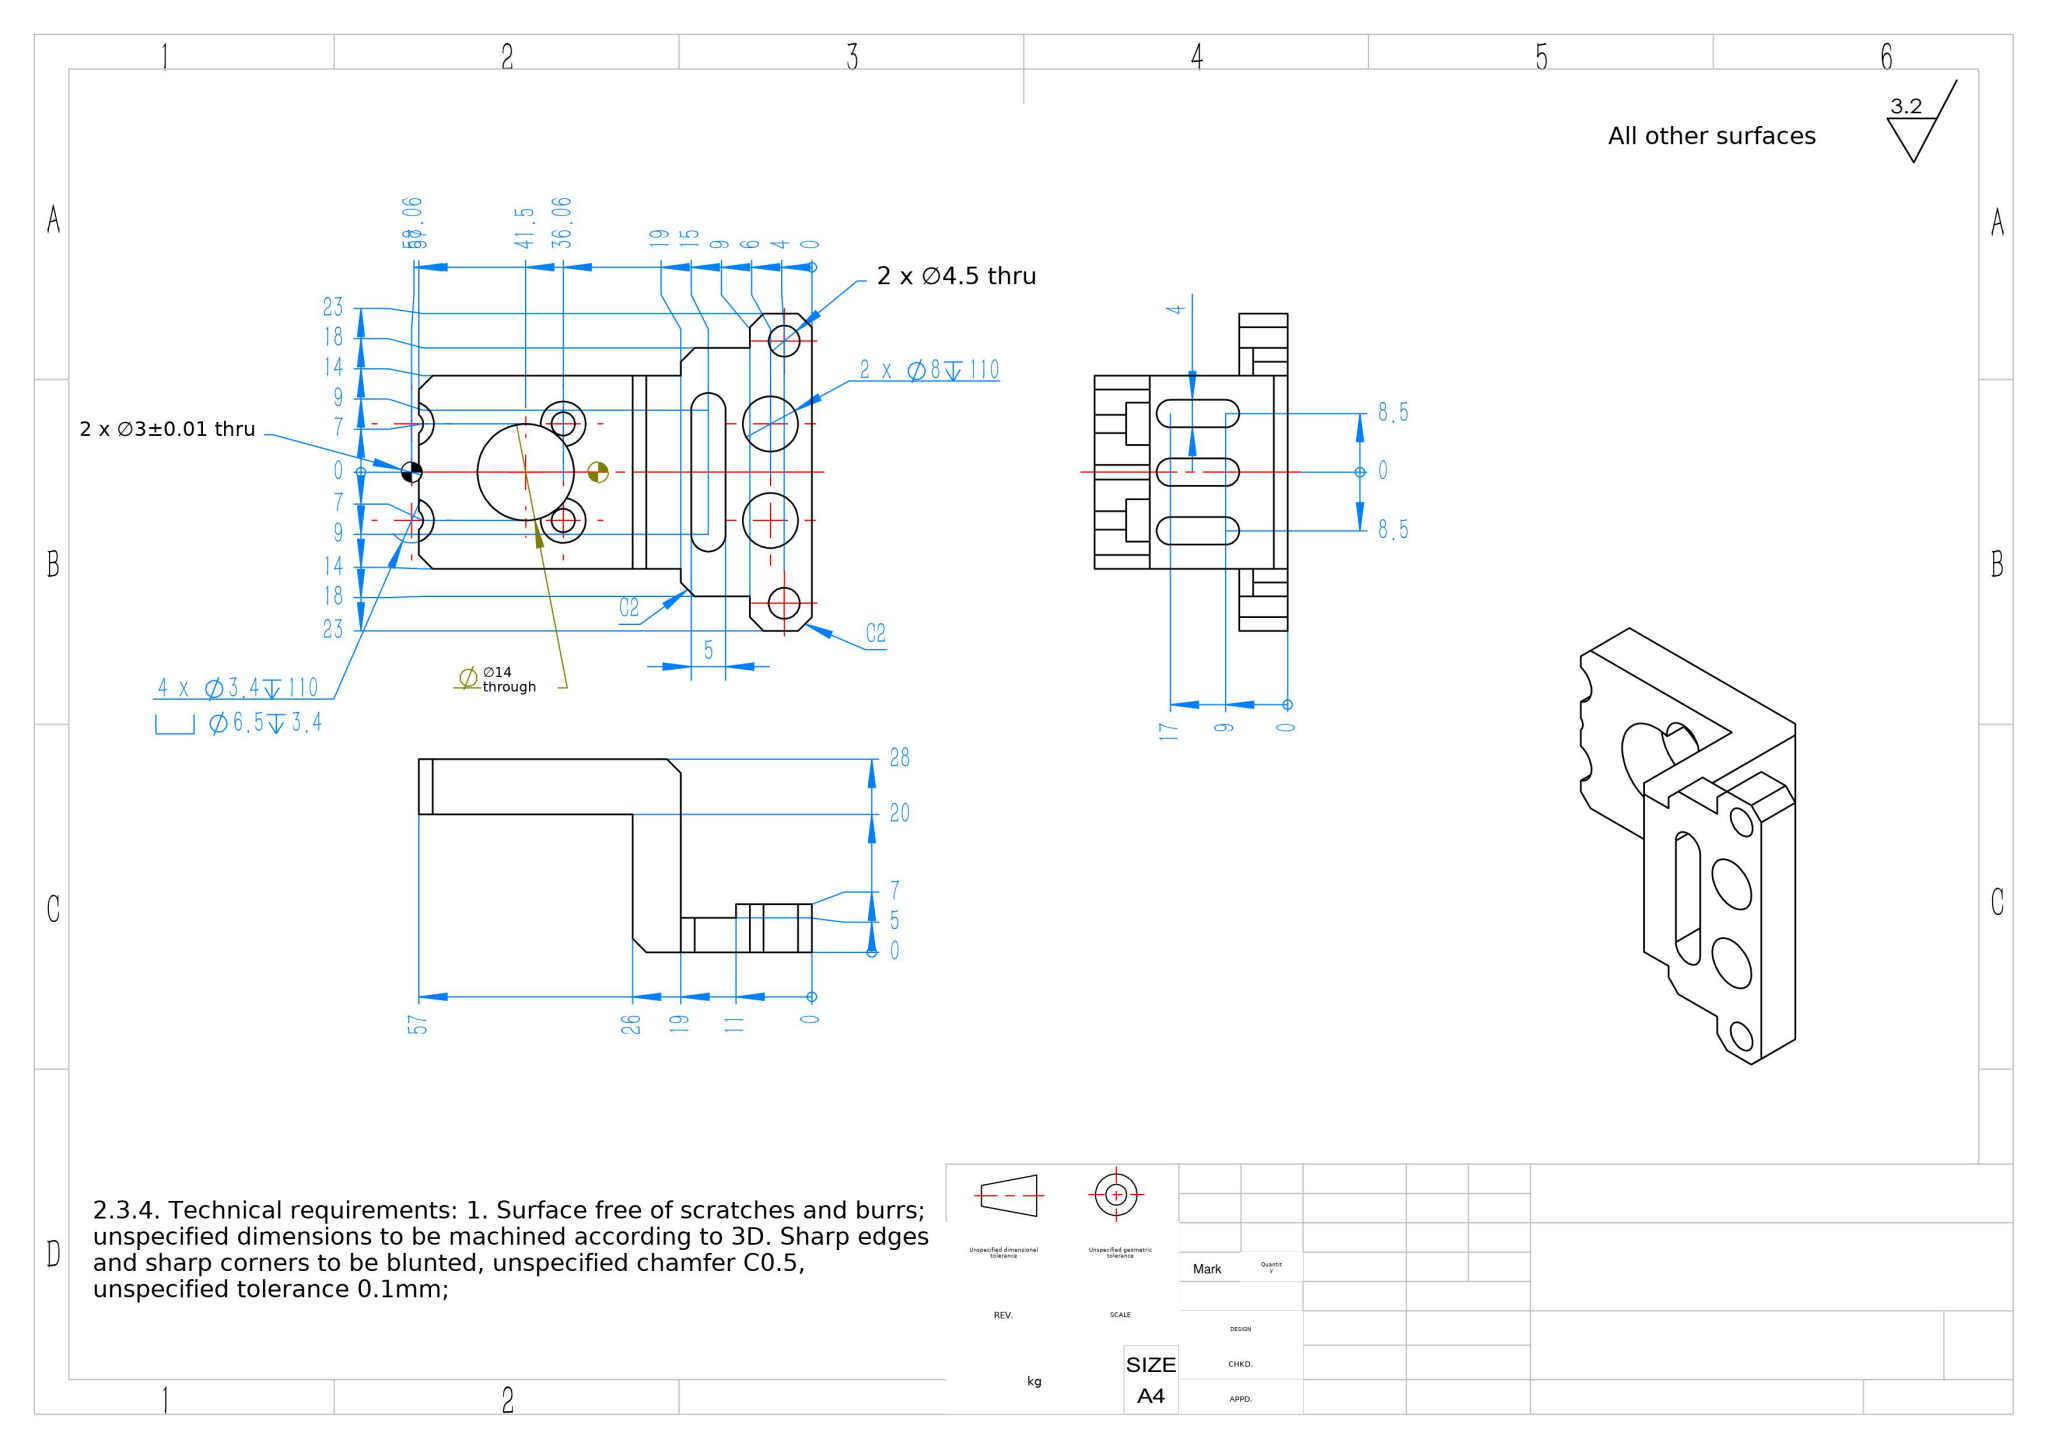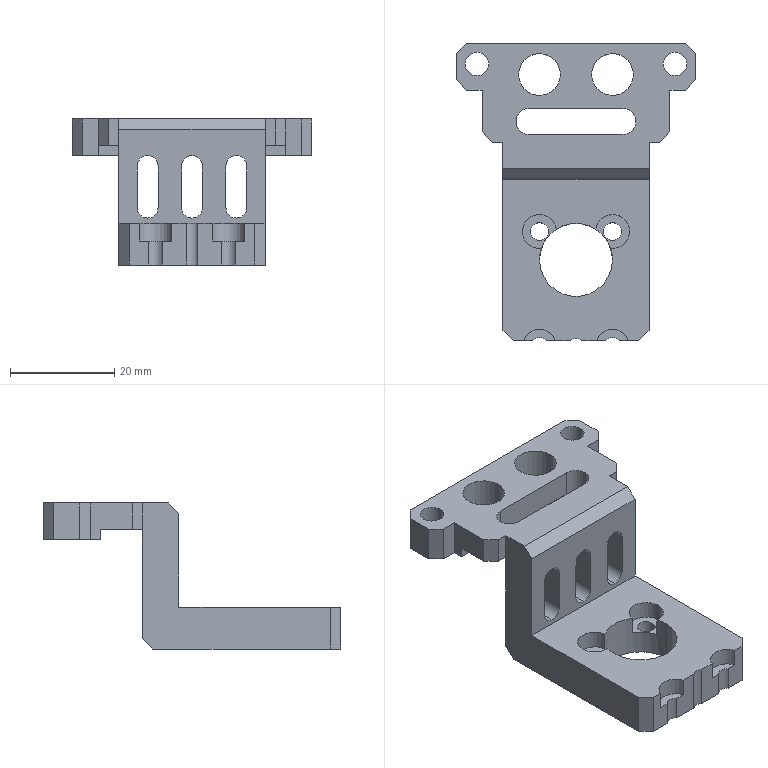Part | SolidWorks | mm | 1 solid | 79 faces | box 46 x 57 x 28 mm | volume 13050 mm3 | plane 45 | cylinder 34 | commonest cylinder face diameters 4 x9 3.4 x6 6.5 x5 8 x4 4.5 x4 5 x3 14 x2 3 x1